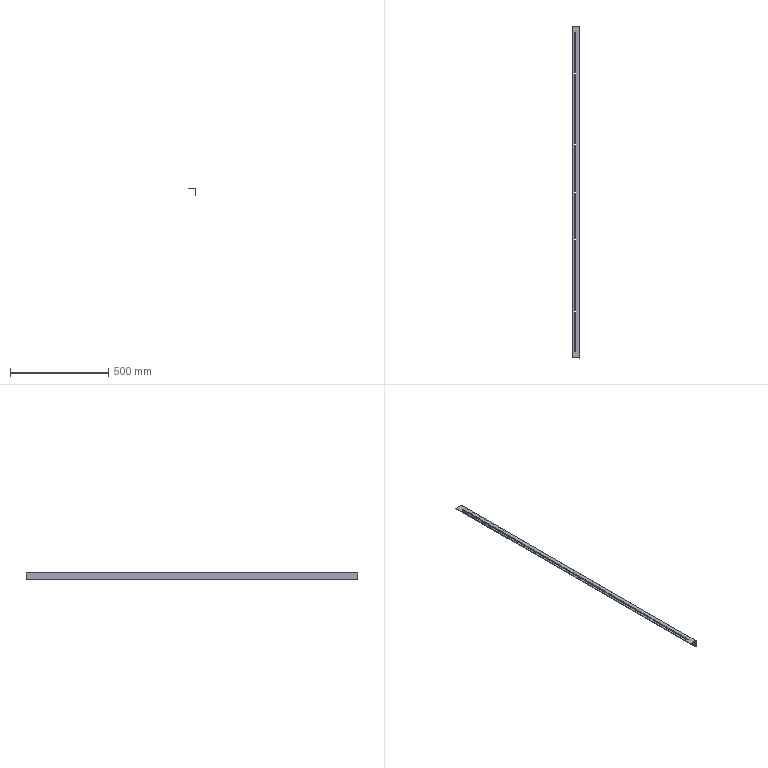Component | SolidWorks | UniversalAngleIron38x38x1690-1 | 1 solid | 108 faces | box 38 x 1690 x 38 mm | volume 335140 mm3 | plane 58 | cylinder 50 | commonest cylinder face diameters 8 x50
build123d program:
from build123d import *

# Parameters (mm, degrees)
EXTRUDE_THIN1_DEPTH = 845
EXTRUDE1_REACH      = 848.707
LPATTERN1_COUNT     = 13
LPATTERN1_PITCH     = 65
LPATTERN1_COL_COUNT = 13
LPATTERN1_COL_PITCH = 65


with BuildPart() as part:
    # Sketch1 → Extrude-Thin1 (new, symmetric)
    with BuildSketch(Plane(origin=(0, 0, 0), x_dir=(1, 0, 0), z_dir=(0, 1, 0))):
        Polygon((0, 38), (0, 0), (-38, 0), (-38, 3), (-3, 3), (-3, 38), align=None)
    extrude(amount=EXTRUDE_THIN1_DEPTH, both=True)

    # Sketch2 → Extrude1 (cut, up to next)
    with BuildSketch(Plane.XY, mode=Mode.PRIVATE) as extrude1_sk1:
        with BuildLine():
            Line((-20, 26), (-20, -26))
            ThreePointArc((-20, -26), (-24, -30), (-28, -26))
            Line((-28, -26), (-28, 26))
            ThreePointArc((-28, 26), (-24, 30), (-20, 26))
        make_face()
    extrude1_tool1 = extrude(extrude1_sk1.sketch, amount=-EXTRUDE1_REACH, mode=Mode.PRIVATE) & part.part
    extrude1 = extrude1_tool1.solids().sort_by_distance((-24, 0, 0))[0]
    add(extrude1, mode=Mode.SUBTRACT)

    # LPattern1: Extrude1 ×13
    with Locations(*[(0, i * LPATTERN1_PITCH, 0) for i in range(1, LPATTERN1_COUNT)]):
        add(extrude1, mode=Mode.SUBTRACT)

    # LPattern1 col: Extrude1 ×13
    with Locations(*[(0, -i * LPATTERN1_COL_PITCH, 0) for i in range(1, LPATTERN1_COL_COUNT)]):
        add(extrude1, mode=Mode.SUBTRACT)


solid = part.part

# Placed as in the assembly
solid = solid.moved(Location((495.8, 848, -105), (0, 0, 0)))